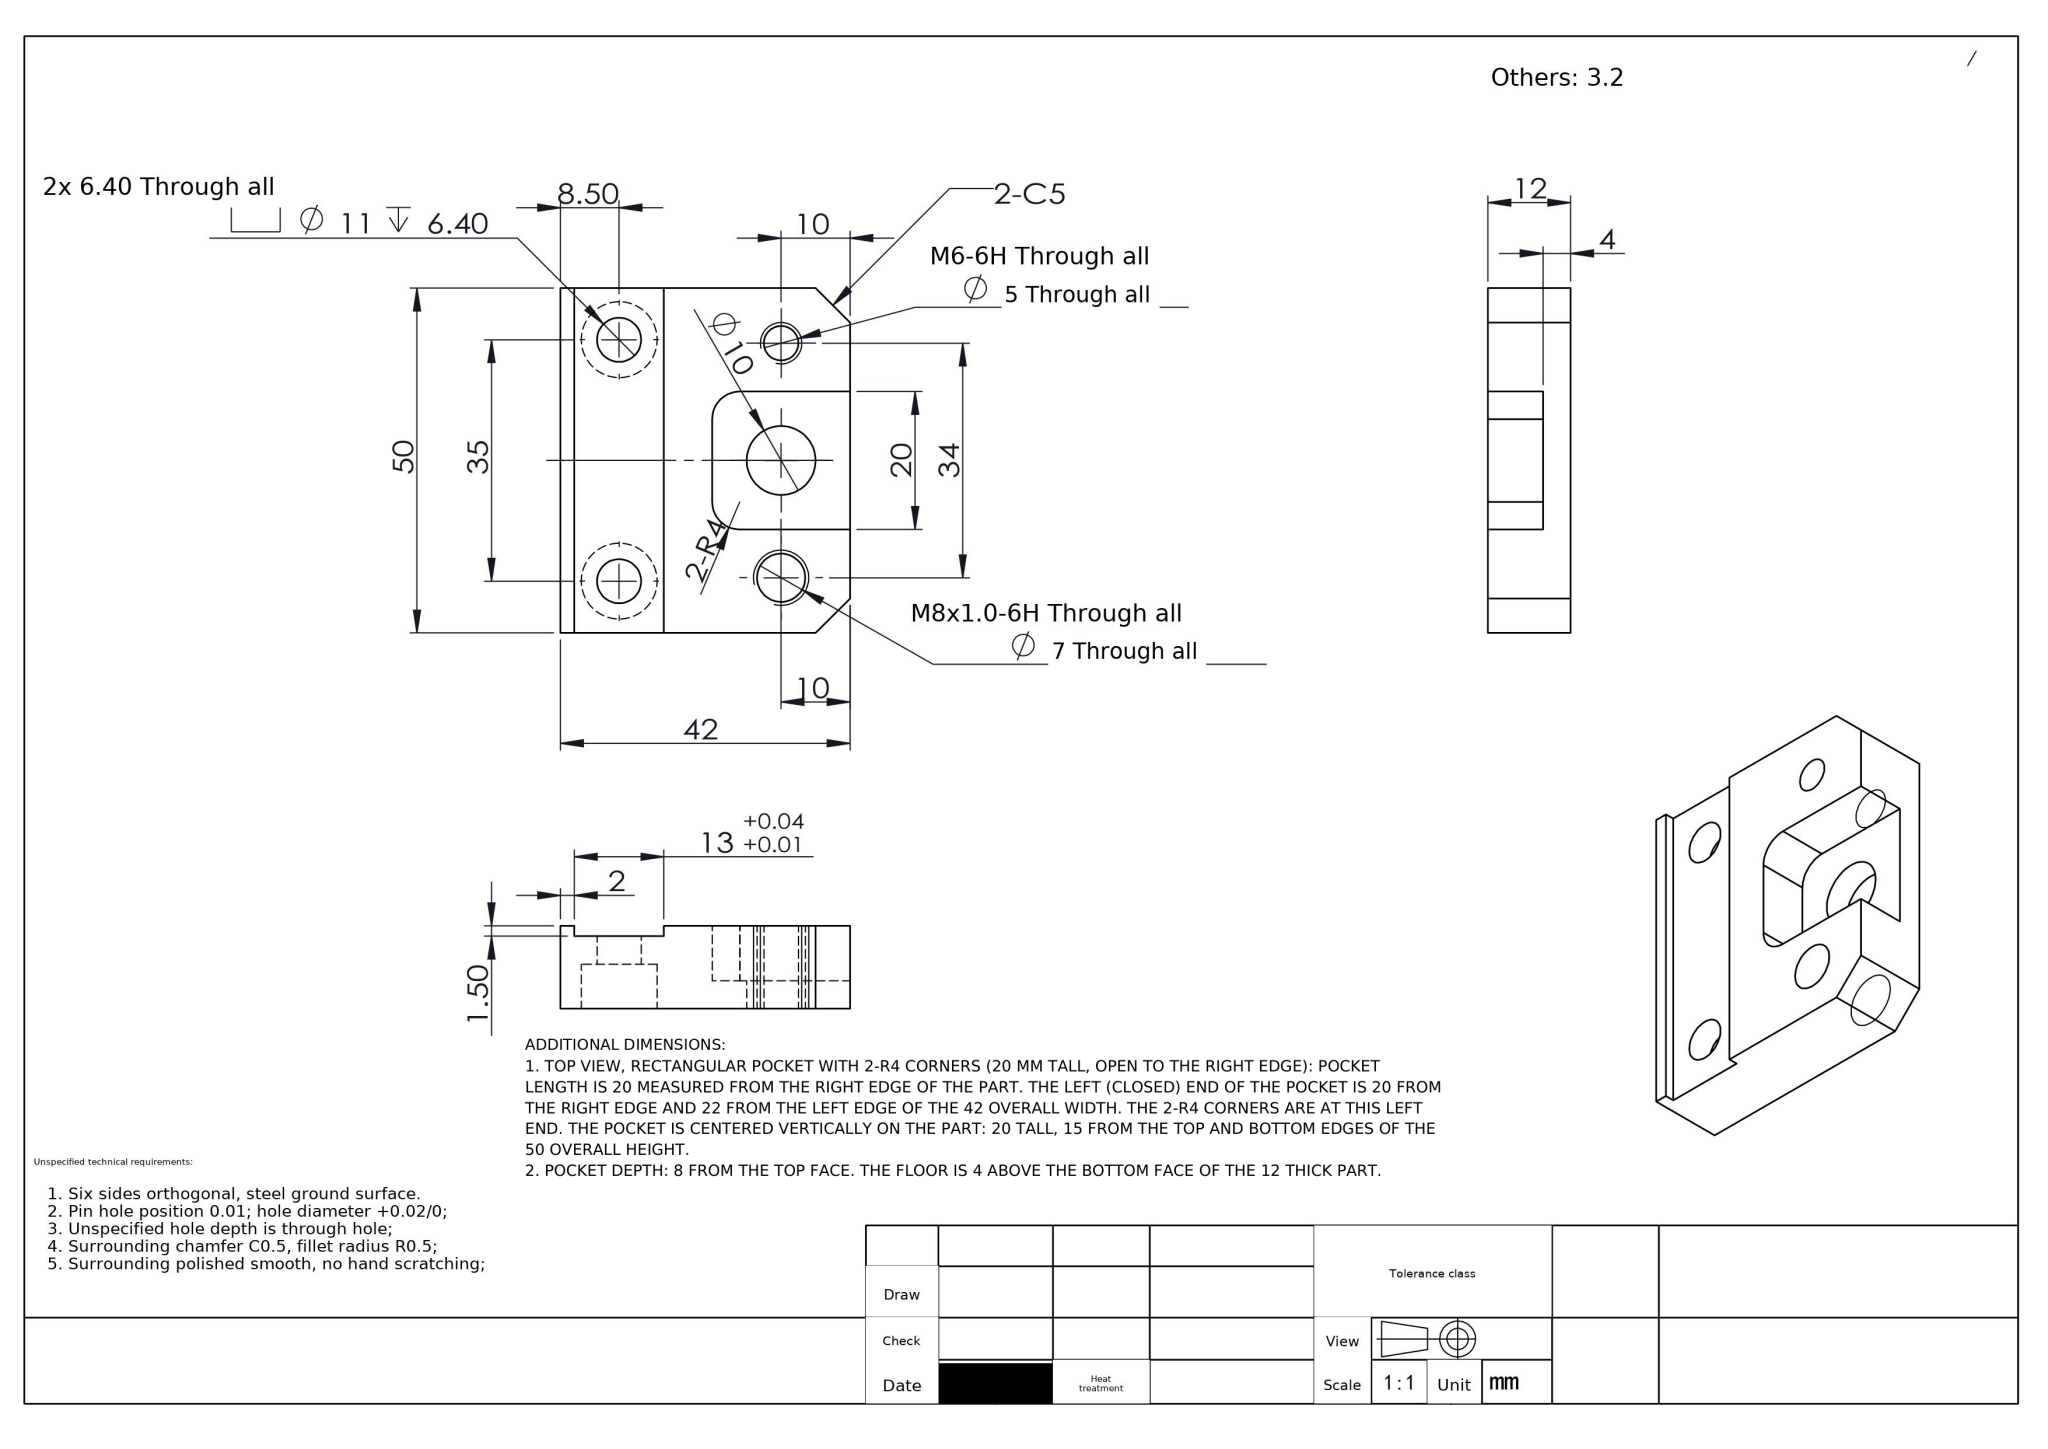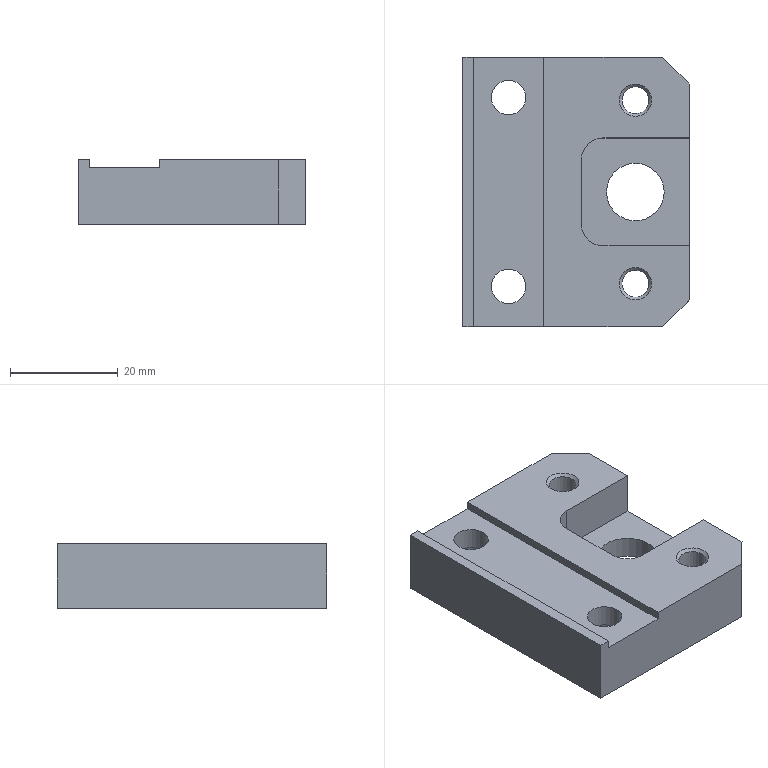Part | NX | mm | Hooked Multi-Bore Mounting Plate | 1 solid | 31 faces | box 42 x 50.01 x 12.01 mm | volume 18460 mm3 | plane 18 | cylinder 9 | cone 4 | commonest cylinder face diameters 6.4 x2 11 x2 8 x2 5 x2 10.7 x1